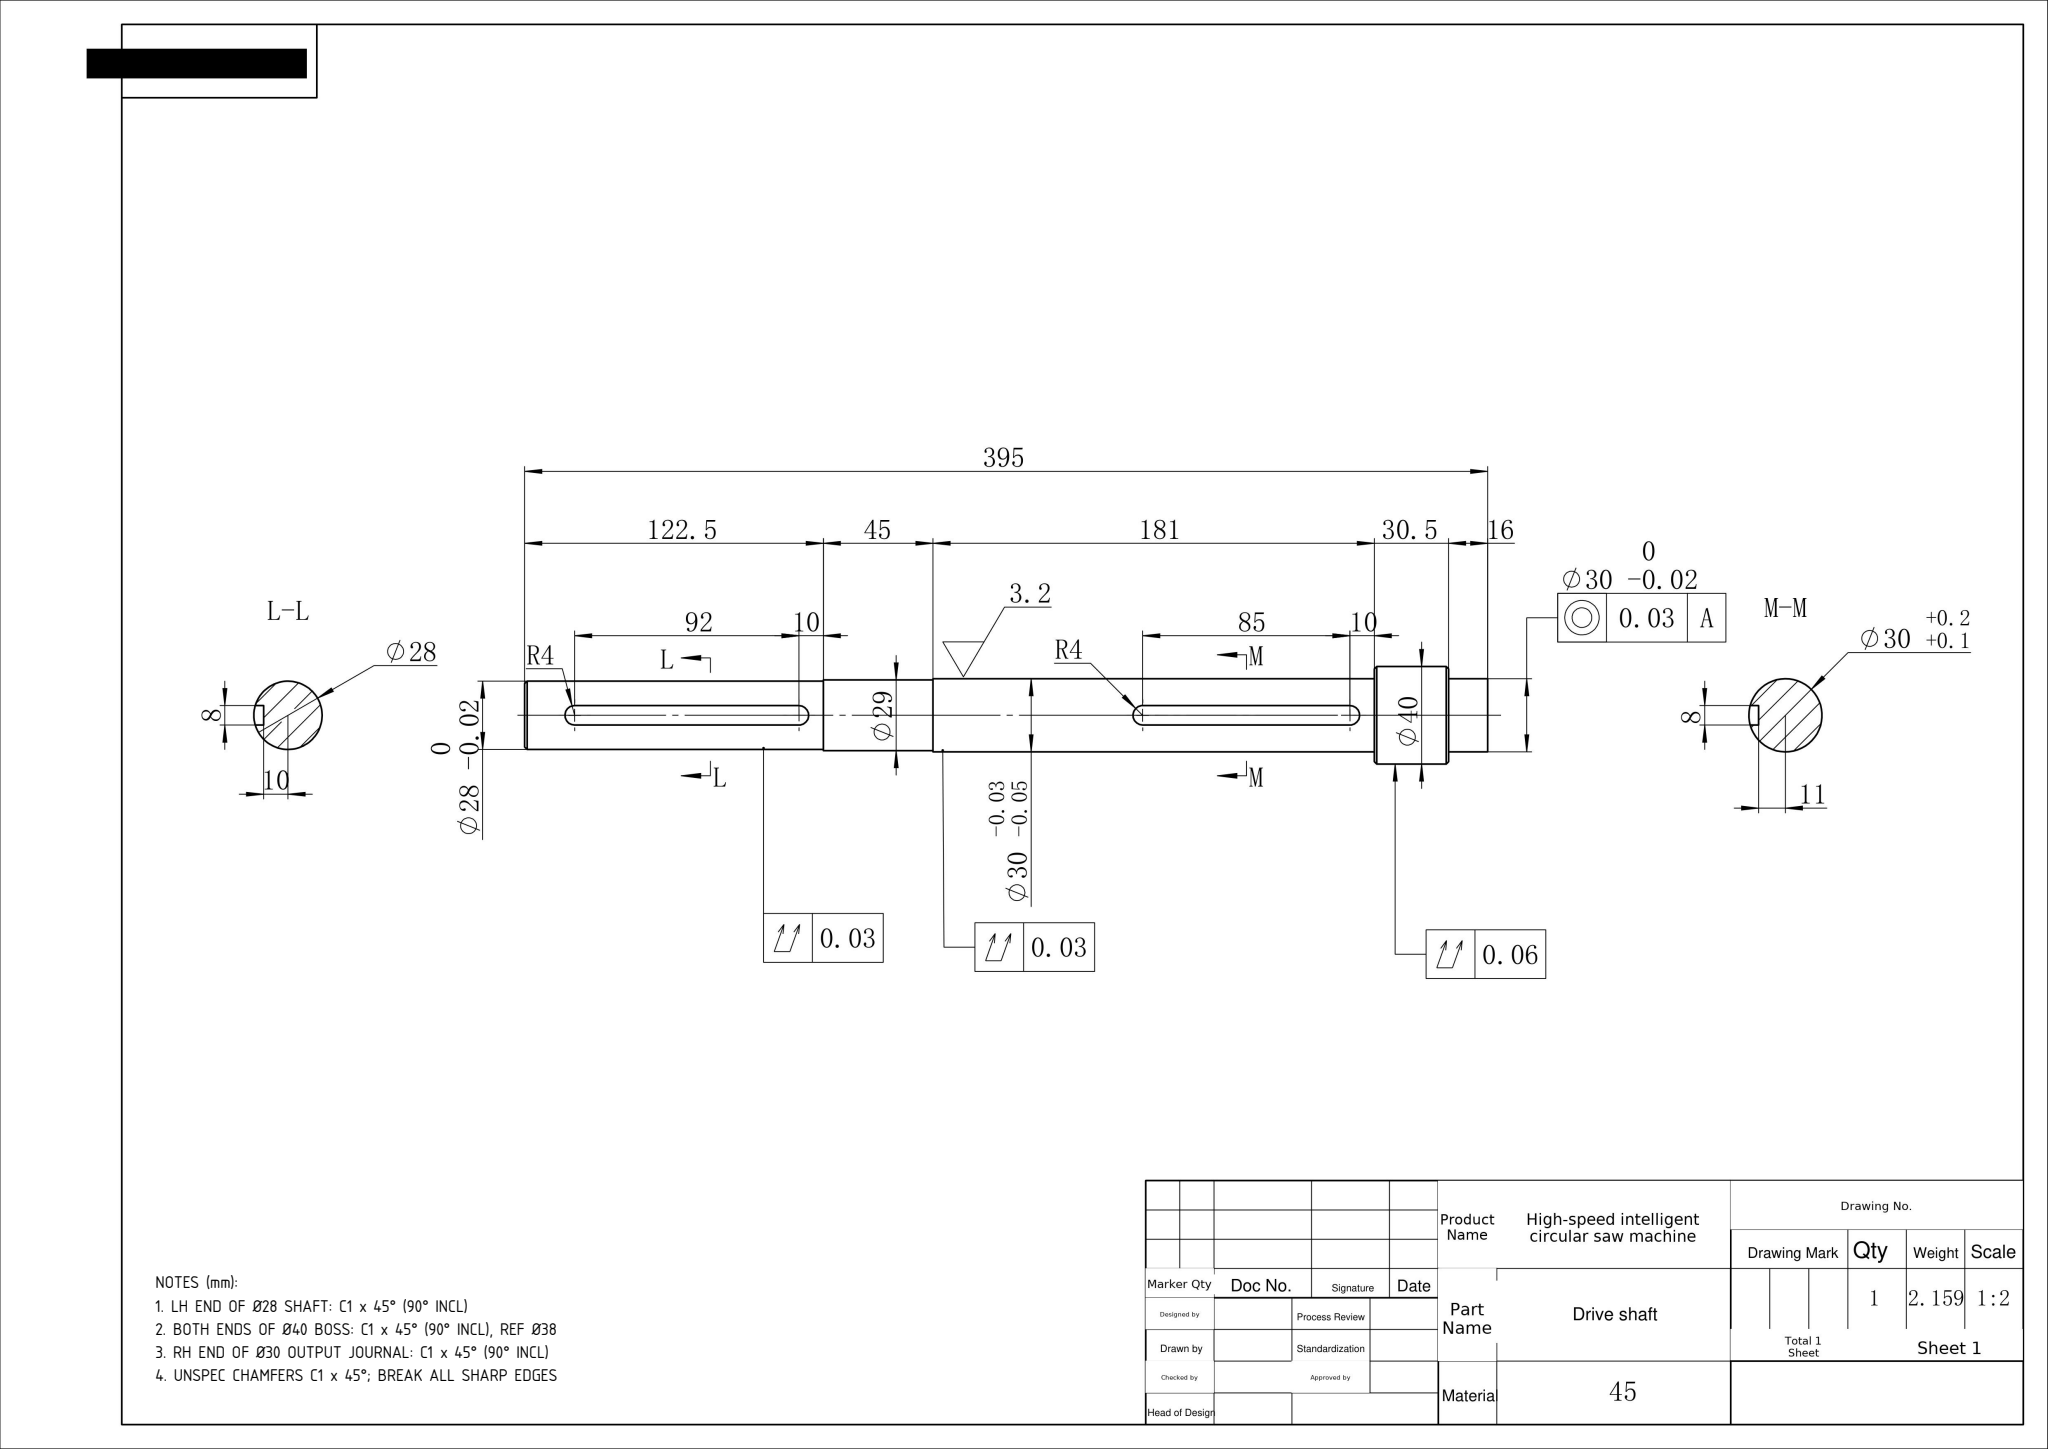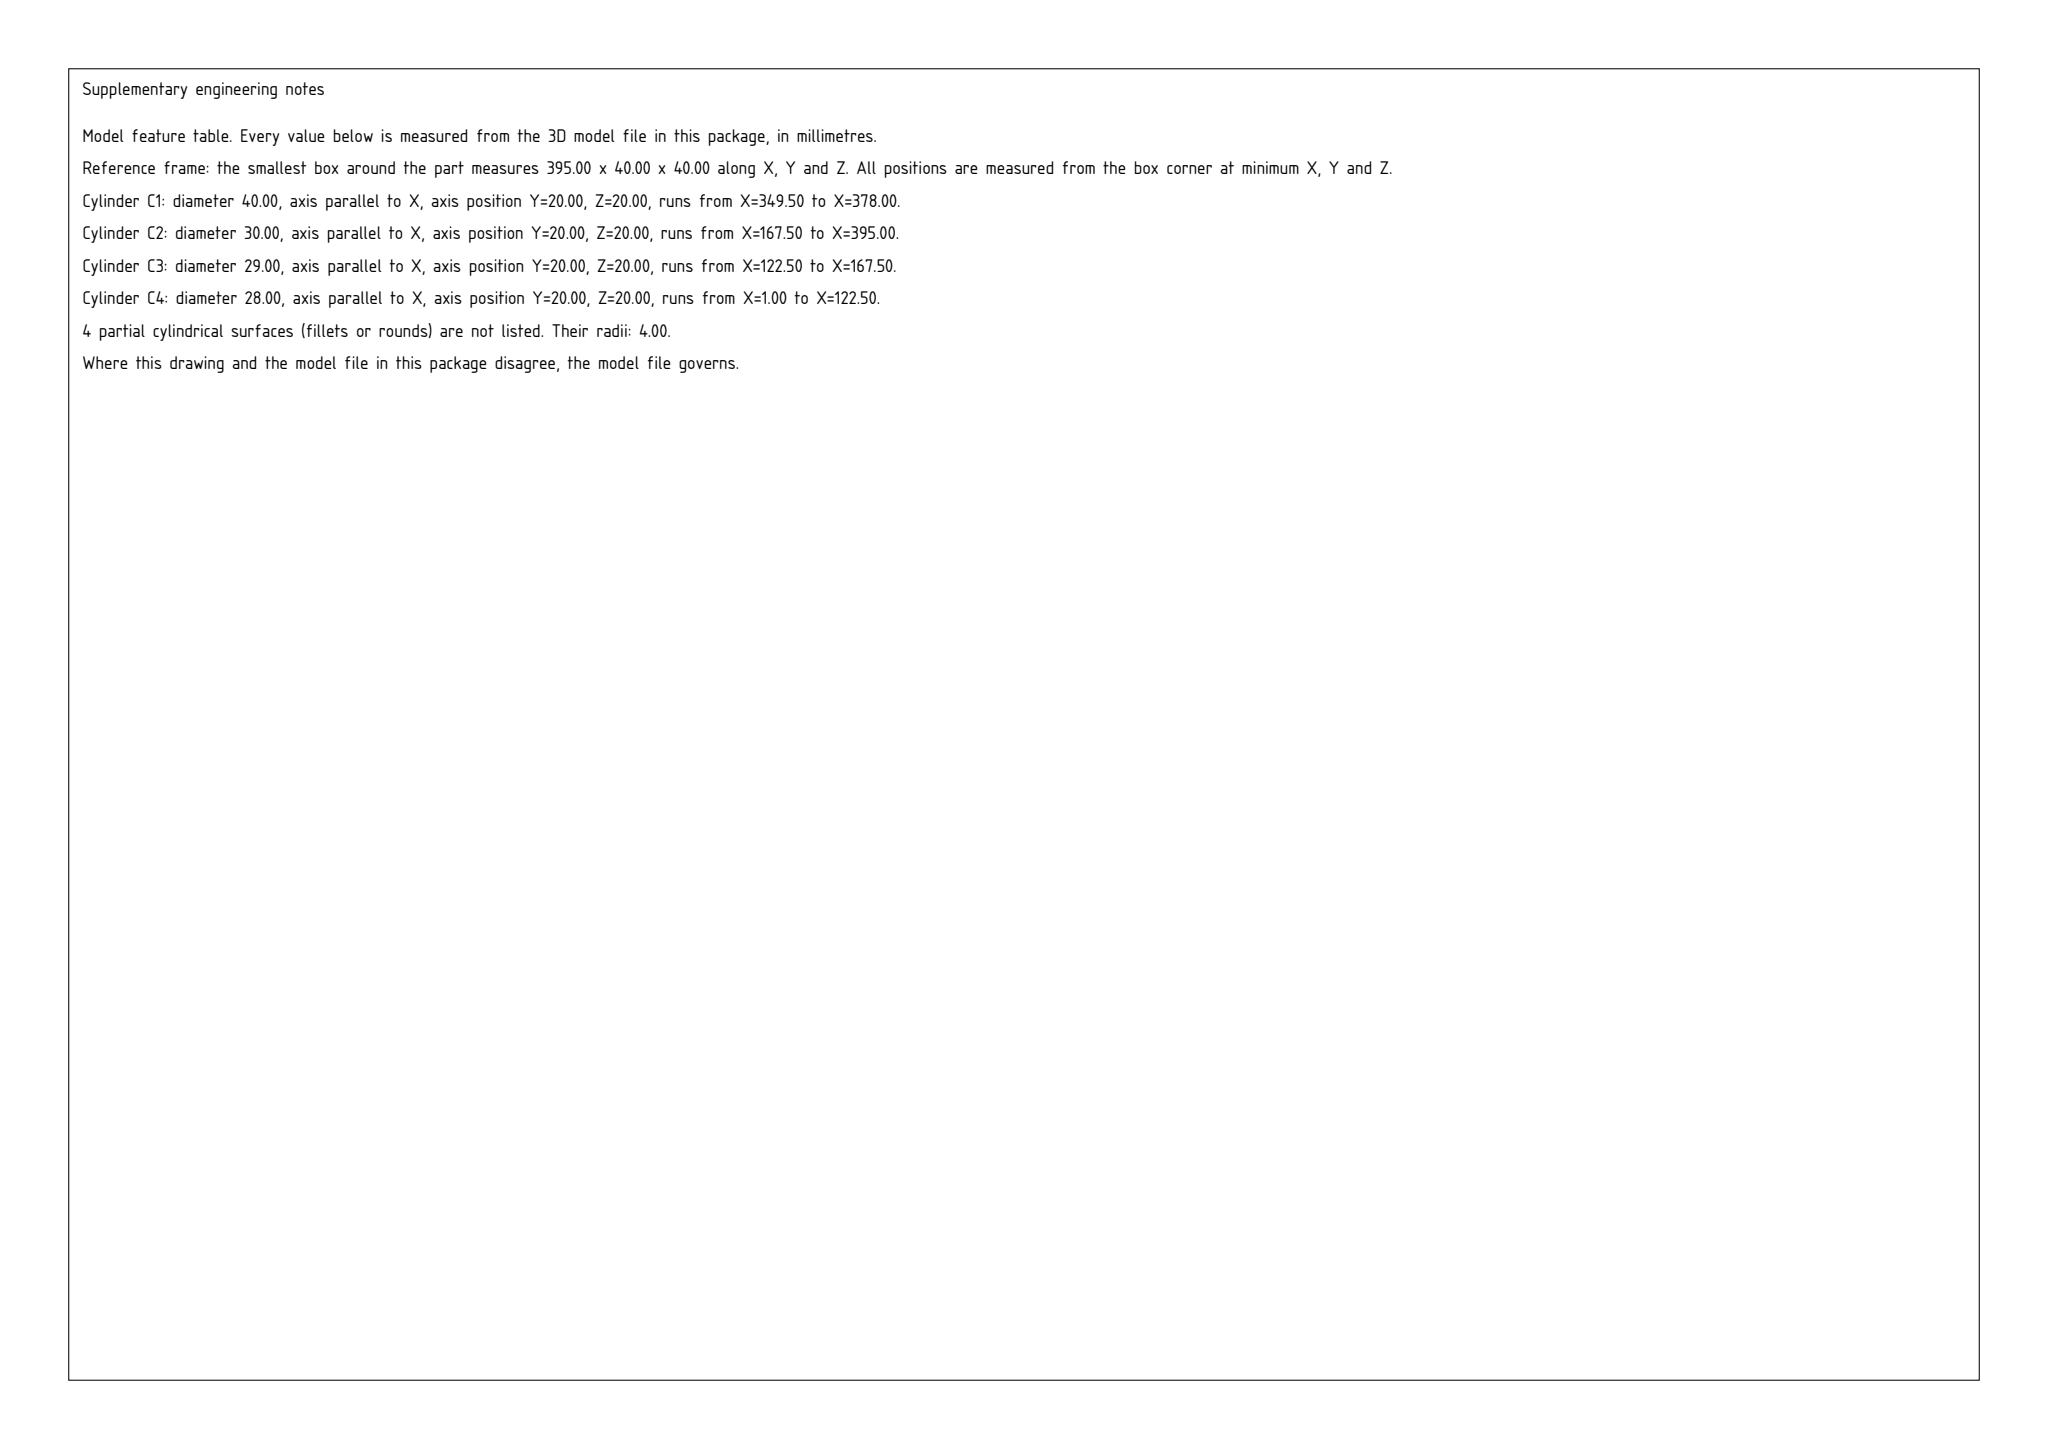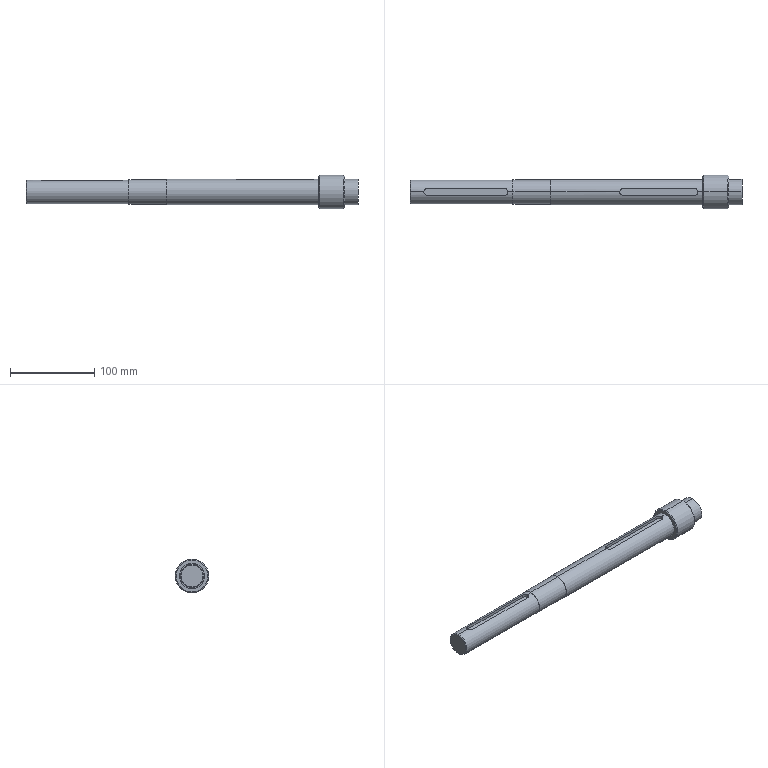Part | SolidWorks | mm | 1 solid | 34 faces | box 395 x 40 x 40 mm | volume 276777 mm3 | cylinder 16 | plane 12 | cone 6 | commonest cylinder face diameters 8 x6 30 x4 28 x2 40 x2 29 x2
Drawing notes:
LH END OF Ø28 SHAFT: C1 x 45° (90° INCL) | from the solid: cones[90.0,26.0] on Ø28 cyl at x=0 => 1mm x 45° chamfer
BOTH ENDS OF Ø40 BOSS: C1 x 45° (90° INCL), REF Ø38 | from the solid: cones[90.0,38.0] & [90.0,40.0] at Ø40 cyl x=348.5-379.0
RH END OF Ø30 OUTPUT JOURNAL: C1 x 45° (90° INCL) | from the solid: 90° cone at x=395 end of Ø30 x 16 long journal
UNSPEC CHAMFERS C1 x 45°; BREAK ALL SHARP EDGES | from the solid: all cones in STEP are 90° included, 1mm leg; no fillet_radii
build123d program:
from build123d import *

# Parameters (mm, degrees)
CHAMFER1_SIZE      = 1
CUT_EXTRUDE1_START = 15
CUT_EXTRUDE1_DEPTH = 4
CUT_EXTRUDE2_START = 14
CUT_EXTRUDE2_DEPTH = 4


with BuildPart() as part:
    # Sketch1 → Revolve1 (revolve)
    with BuildSketch(Plane.XY, mode=Mode.PRIVATE) as revolve1_sk:
        Polygon((-227.5, 15), (-227.5, 14.5), (-272.5, 14.5), (-272.5, 14), (-395, 14), (-395, 0), (0, 0), (0, 15), (-16, 15), (-16, 20), (-46.5, 20), (-46.5, 15), align=None)
    revolve(revolve1_sk.sketch.rotate(Axis((-395, 0, 0), (1, 0, 0)), 90), axis=Axis((-395, 0, 0), (1, 0, 0)))

    # Chamfer1
    chamfer1_edges = [part.edges().sort_by_distance(p)[0] for p in [
        (-16, 0, -20),
        (-46.5, 0, -20),
        (-395, 0, -14),
    ]]
    chamfer(chamfer1_edges, length=CHAMFER1_SIZE)

    # Sketch2 → Cut-Extrude1 (cut)
    with BuildSketch(Plane.XY.offset(CUT_EXTRUDE1_START)):
        with BuildLine():
            Line((-141.5, 4), (-56.5, 4))
            ThreePointArc((-56.5, 4), (-52.5, 0), (-56.5, -4))
            Line((-56.5, -4), (-141.5, -4))
            ThreePointArc((-141.5, -4), (-145.5, 0), (-141.5, 4))
        make_face()
    extrude(amount=-CUT_EXTRUDE1_DEPTH, mode=Mode.SUBTRACT)

    # Sketch3 → Cut-Extrude2 (cut)
    with BuildSketch(Plane.XY.offset(CUT_EXTRUDE2_START)):
        with BuildLine():
            Line((-282.5, -4), (-374.5, -4))
            ThreePointArc((-374.5, -4), (-378.5, 0), (-374.5, 4))
            Line((-374.5, 4), (-282.5, 4))
            ThreePointArc((-282.5, 4), (-278.5, 0), (-282.5, -4))
        make_face()
    extrude(amount=-CUT_EXTRUDE2_DEPTH, mode=Mode.SUBTRACT)


solid = part.part